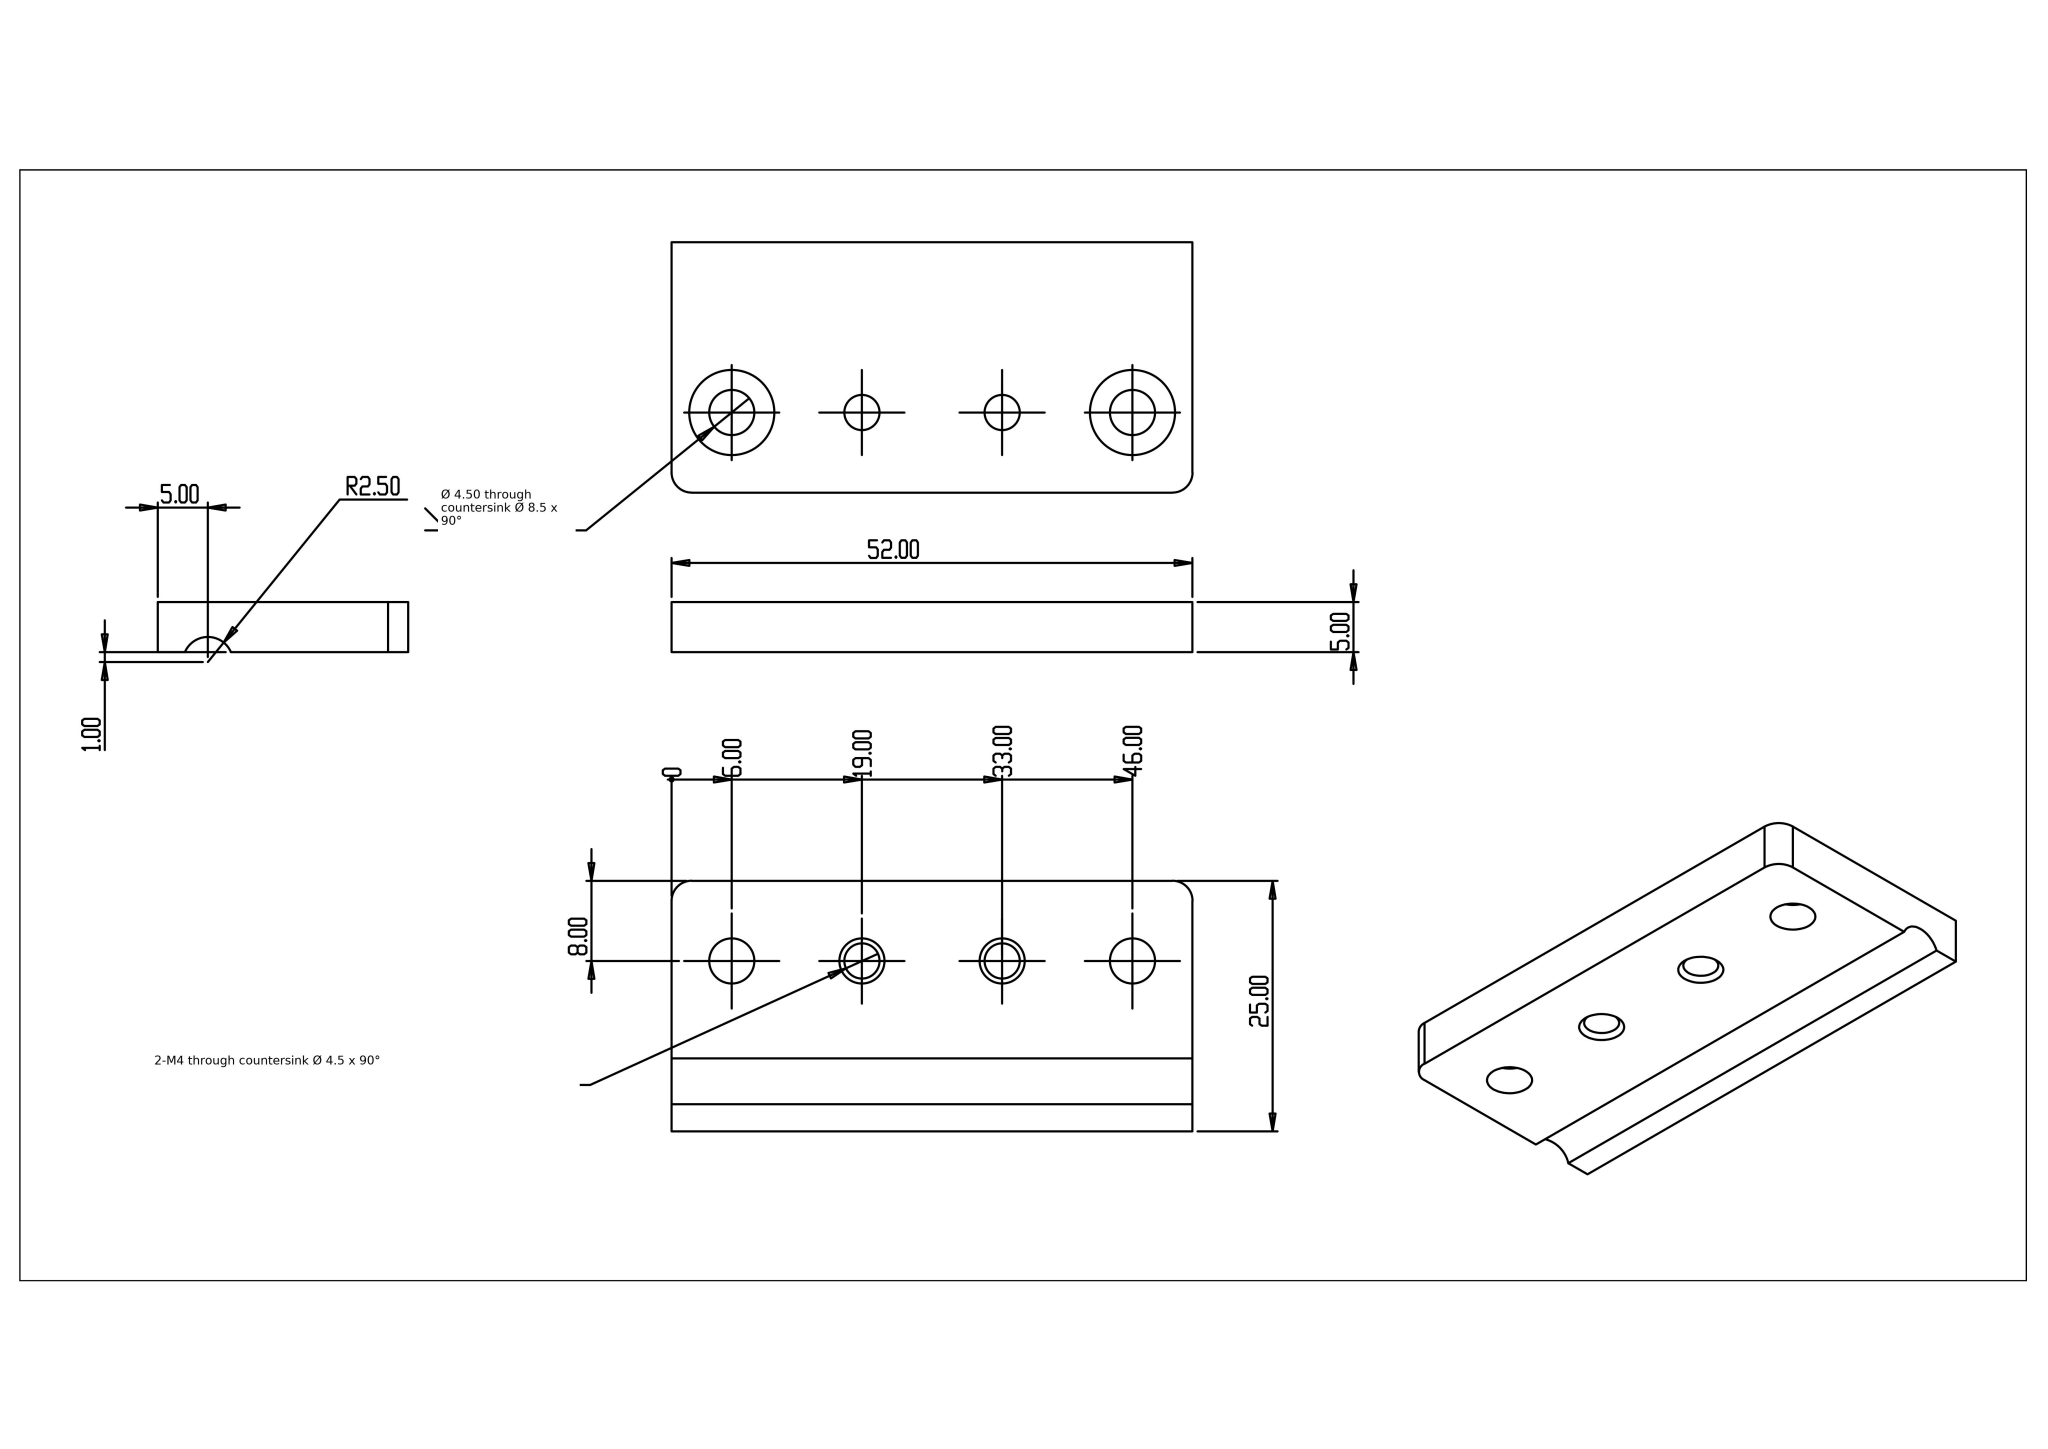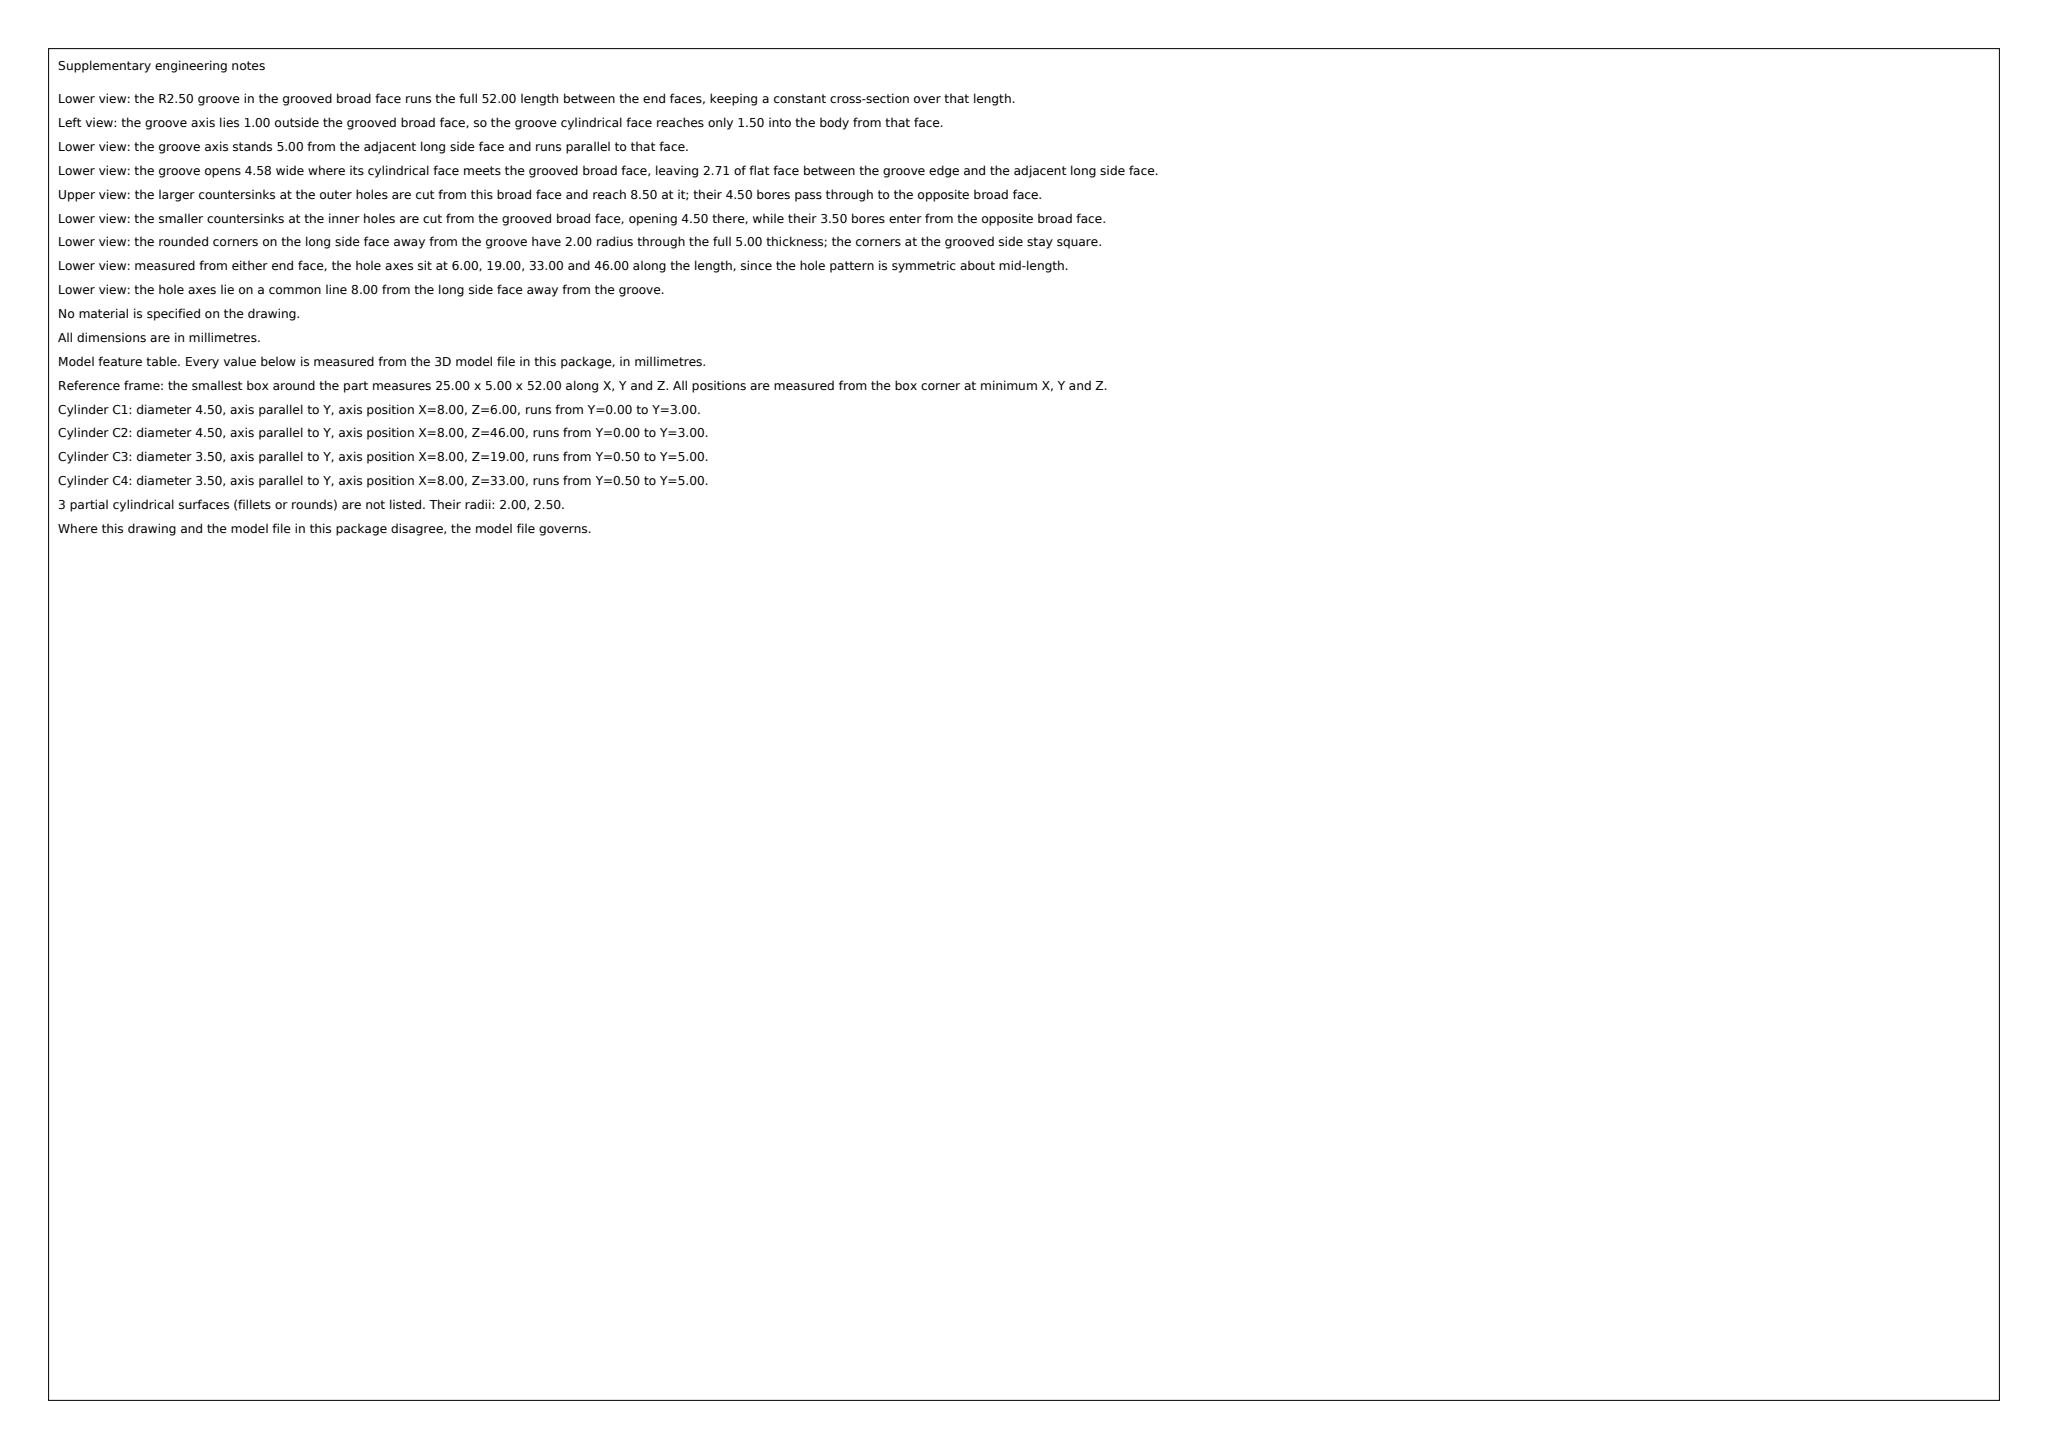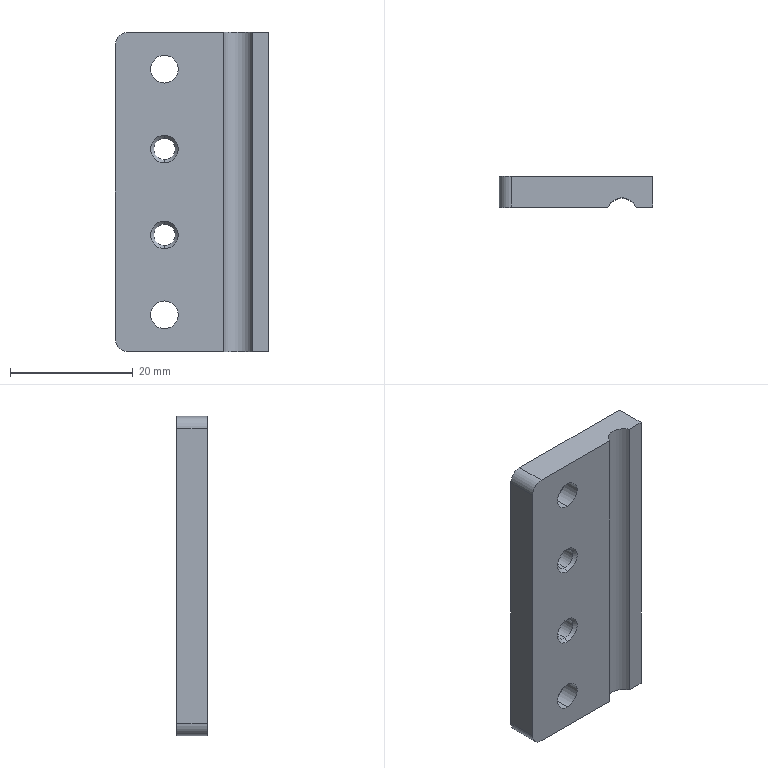Part | SolidWorks | mm | 1 solid | 26 faces | box 25 x 5 x 52 mm | volume 5902 mm3 | cylinder 11 | cone 8 | plane 7 | commonest cylinder face diameters 4.5 x4 3.5 x4 4 x2 5 x1
Drawing notes:
2X Ø4.50 THRU, C'SINK Ø8.5 X 90° AT 6.00 & 46.00 | from the solid: cylinders Ø4.5 axis y at z=6.0 and z=46.0, x=8.0 (2 instances each); cones 90° ref dia 4.5
build123d program:
from build123d import *

# Parameters (mm, degrees)
BOSS_EXTRUDE1_DEPTH = 52
CUT_EXTRUDE1_REACH  = 55.715
SKETCH2_R           = 1.75
CHAMFER1_SIZE       = 0.5
CHAMFER2_SIZE       = 2


with BuildPart() as part:
    # Sketch1 → Boss-Extrude1 (new body)
    with BuildSketch(Plane.XY):
        with BuildLine():
            Line((12.5, -2.5), (12.5, 2.5))
            Line((12.5, 2.5), (10.5, 2.5))
            Line((10.5, 2.5), (-10.5, 2.5))
            Line((-10.5, 2.5), (-12.5, 2.5))
            Line((-12.5, 2.5), (-12.5, -2.5))
            Line((-12.5, -2.5), (-10.5, -2.5))
            Line((-10.5, -2.5), (5.209, -2.5))
            ThreePointArc((5.209, -2.5), (7.5, -1), (9.791, -2.5))
            Line((9.791, -2.5), (10.5, -2.5))
            Line((10.5, -2.5), (12.5, -2.5))
        make_face()
    extrude(amount=BOSS_EXTRUDE1_DEPTH)

    # Sketch2 → Cut-Extrude1 (cut, up to next)
    with BuildSketch(Plane.XZ.offset(2.5), mode=Mode.PRIVATE) as cut_extrude1_sk1:
        with Locations(Location((-4.5, 33, 0), (0, 0, 270))):
            Circle(SKETCH2_R)
    cut_extrude1_tool1 = extrude(cut_extrude1_sk1.sketch, amount=-CUT_EXTRUDE1_REACH, mode=Mode.PRIVATE) & part.part
    # Sketch2 → Cut-Extrude1 (cut, up to next)
    with BuildSketch(Plane.XZ.offset(2.5), mode=Mode.PRIVATE) as cut_extrude1_sk2:
        with Locations(Location((-4.5, 19, 0), (0, 0, 270))):
            Circle(SKETCH2_R)
    cut_extrude1_tool2 = extrude(cut_extrude1_sk2.sketch, amount=-CUT_EXTRUDE1_REACH, mode=Mode.PRIVATE) & part.part
    # Sketch2 → Cut-Extrude1 (cut, up to next)
    with BuildSketch(Plane.XZ.offset(2.5), mode=Mode.PRIVATE) as cut_extrude1_sk3:
        with BuildLine():
            Line((-10.5, 52), (-12.5, 52))
            Line((-12.5, 52), (-12.5, 50))
            ThreePointArc((-12.5, 50), (-11.914, 51.414), (-10.5, 52))
        make_face()
    cut_extrude1_tool3 = extrude(cut_extrude1_sk3.sketch, amount=-CUT_EXTRUDE1_REACH, mode=Mode.PRIVATE) & part.part
    # Sketch2 → Cut-Extrude1 (cut, up to next)
    with BuildSketch(Plane.XZ.offset(2.5), mode=Mode.PRIVATE) as cut_extrude1_sk4:
        with BuildLine():
            Line((-10.5, 0), (-12.5, 0))
            Line((-12.5, 0), (-12.5, 2))
            ThreePointArc((-12.5, 2), (-11.914, 0.5858), (-10.5, 0))
        make_face()
    cut_extrude1_tool4 = extrude(cut_extrude1_sk4.sketch, amount=-CUT_EXTRUDE1_REACH, mode=Mode.PRIVATE) & part.part
    # Sketch2 → Cut-Extrude1 (cut, up to next)
    with BuildSketch(Plane.XZ.offset(2.5), mode=Mode.PRIVATE) as cut_extrude1_sk5:
        with BuildLine():
            ThreePointArc((-4.5, 48.25), (-6.75, 46), (-4.5, 43.75))
            ThreePointArc((-4.5, 43.75), (-2.25, 46), (-4.5, 48.25))
        make_face()
    cut_extrude1_tool5 = extrude(cut_extrude1_sk5.sketch, amount=-CUT_EXTRUDE1_REACH, mode=Mode.PRIVATE) & part.part
    # Sketch2 → Cut-Extrude1 (cut, up to next)
    with BuildSketch(Plane.XZ.offset(2.5), mode=Mode.PRIVATE) as cut_extrude1_sk6:
        with BuildLine():
            ThreePointArc((-4.5, 8.25), (-6.75, 6), (-4.5, 3.75))
            ThreePointArc((-4.5, 3.75), (-2.25, 6), (-4.5, 8.25))
        make_face()
    cut_extrude1_tool6 = extrude(cut_extrude1_sk6.sketch, amount=-CUT_EXTRUDE1_REACH, mode=Mode.PRIVATE) & part.part
    add(cut_extrude1_tool1.solids().sort_by_distance((-4.5, -2.5, 33))[0], mode=Mode.SUBTRACT)
    add(cut_extrude1_tool2.solids().sort_by_distance((-4.5, -2.5, 19))[0], mode=Mode.SUBTRACT)
    add(cut_extrude1_tool3.solids().sort_by_distance((-12.053, -2.5, 51.553))[0], mode=Mode.SUBTRACT)
    add(cut_extrude1_tool4.solids().sort_by_distance((-12.053, -2.5, 0.4467))[0], mode=Mode.SUBTRACT)
    add(cut_extrude1_tool5.solids().sort_by_distance((-4.5, -2.5, 46))[0], mode=Mode.SUBTRACT)
    add(cut_extrude1_tool6.solids().sort_by_distance((-4.5, -2.5, 6))[0], mode=Mode.SUBTRACT)

    # Chamfer1
    chamfer1_edges = [part.edges().sort_by_distance(p)[0] for p in [
        (-4.5, -2.5, 34.75),
        (-4.5, -2.5, 20.75),
    ]]
    chamfer(chamfer1_edges, length=CHAMFER1_SIZE)

    # Chamfer2
    chamfer2_edges = [part.edges().sort_by_distance(p)[0] for p in [
        (-4.5, 2.5, 3.75),
        (-4.5, 2.5, 48.25),
    ]]
    chamfer(chamfer2_edges, length=CHAMFER2_SIZE)


solid = part.part